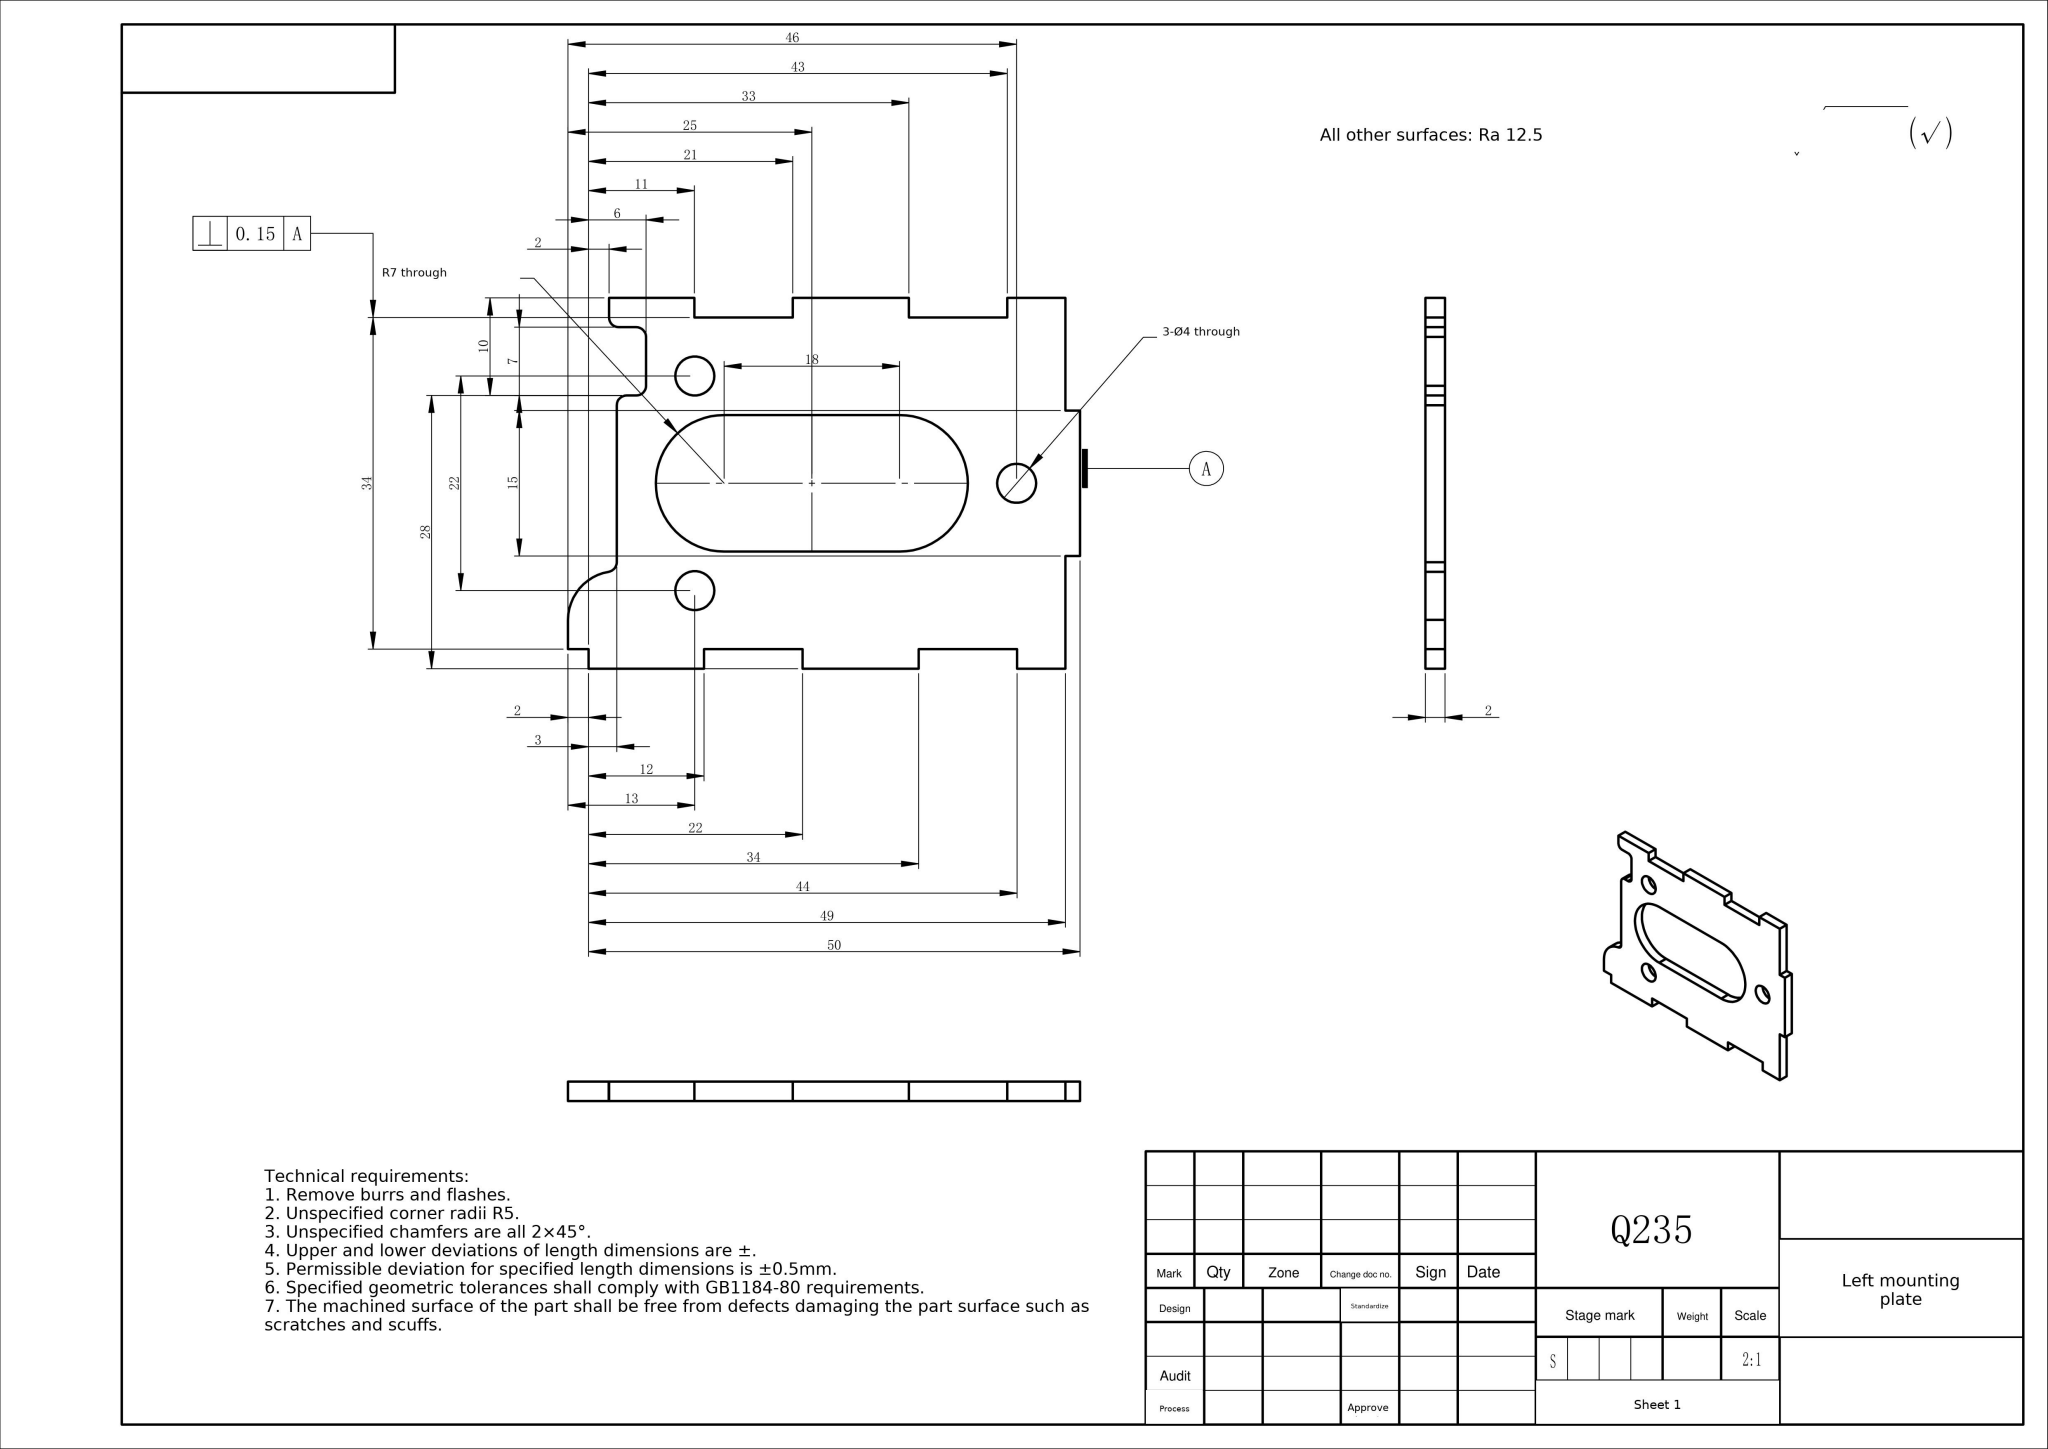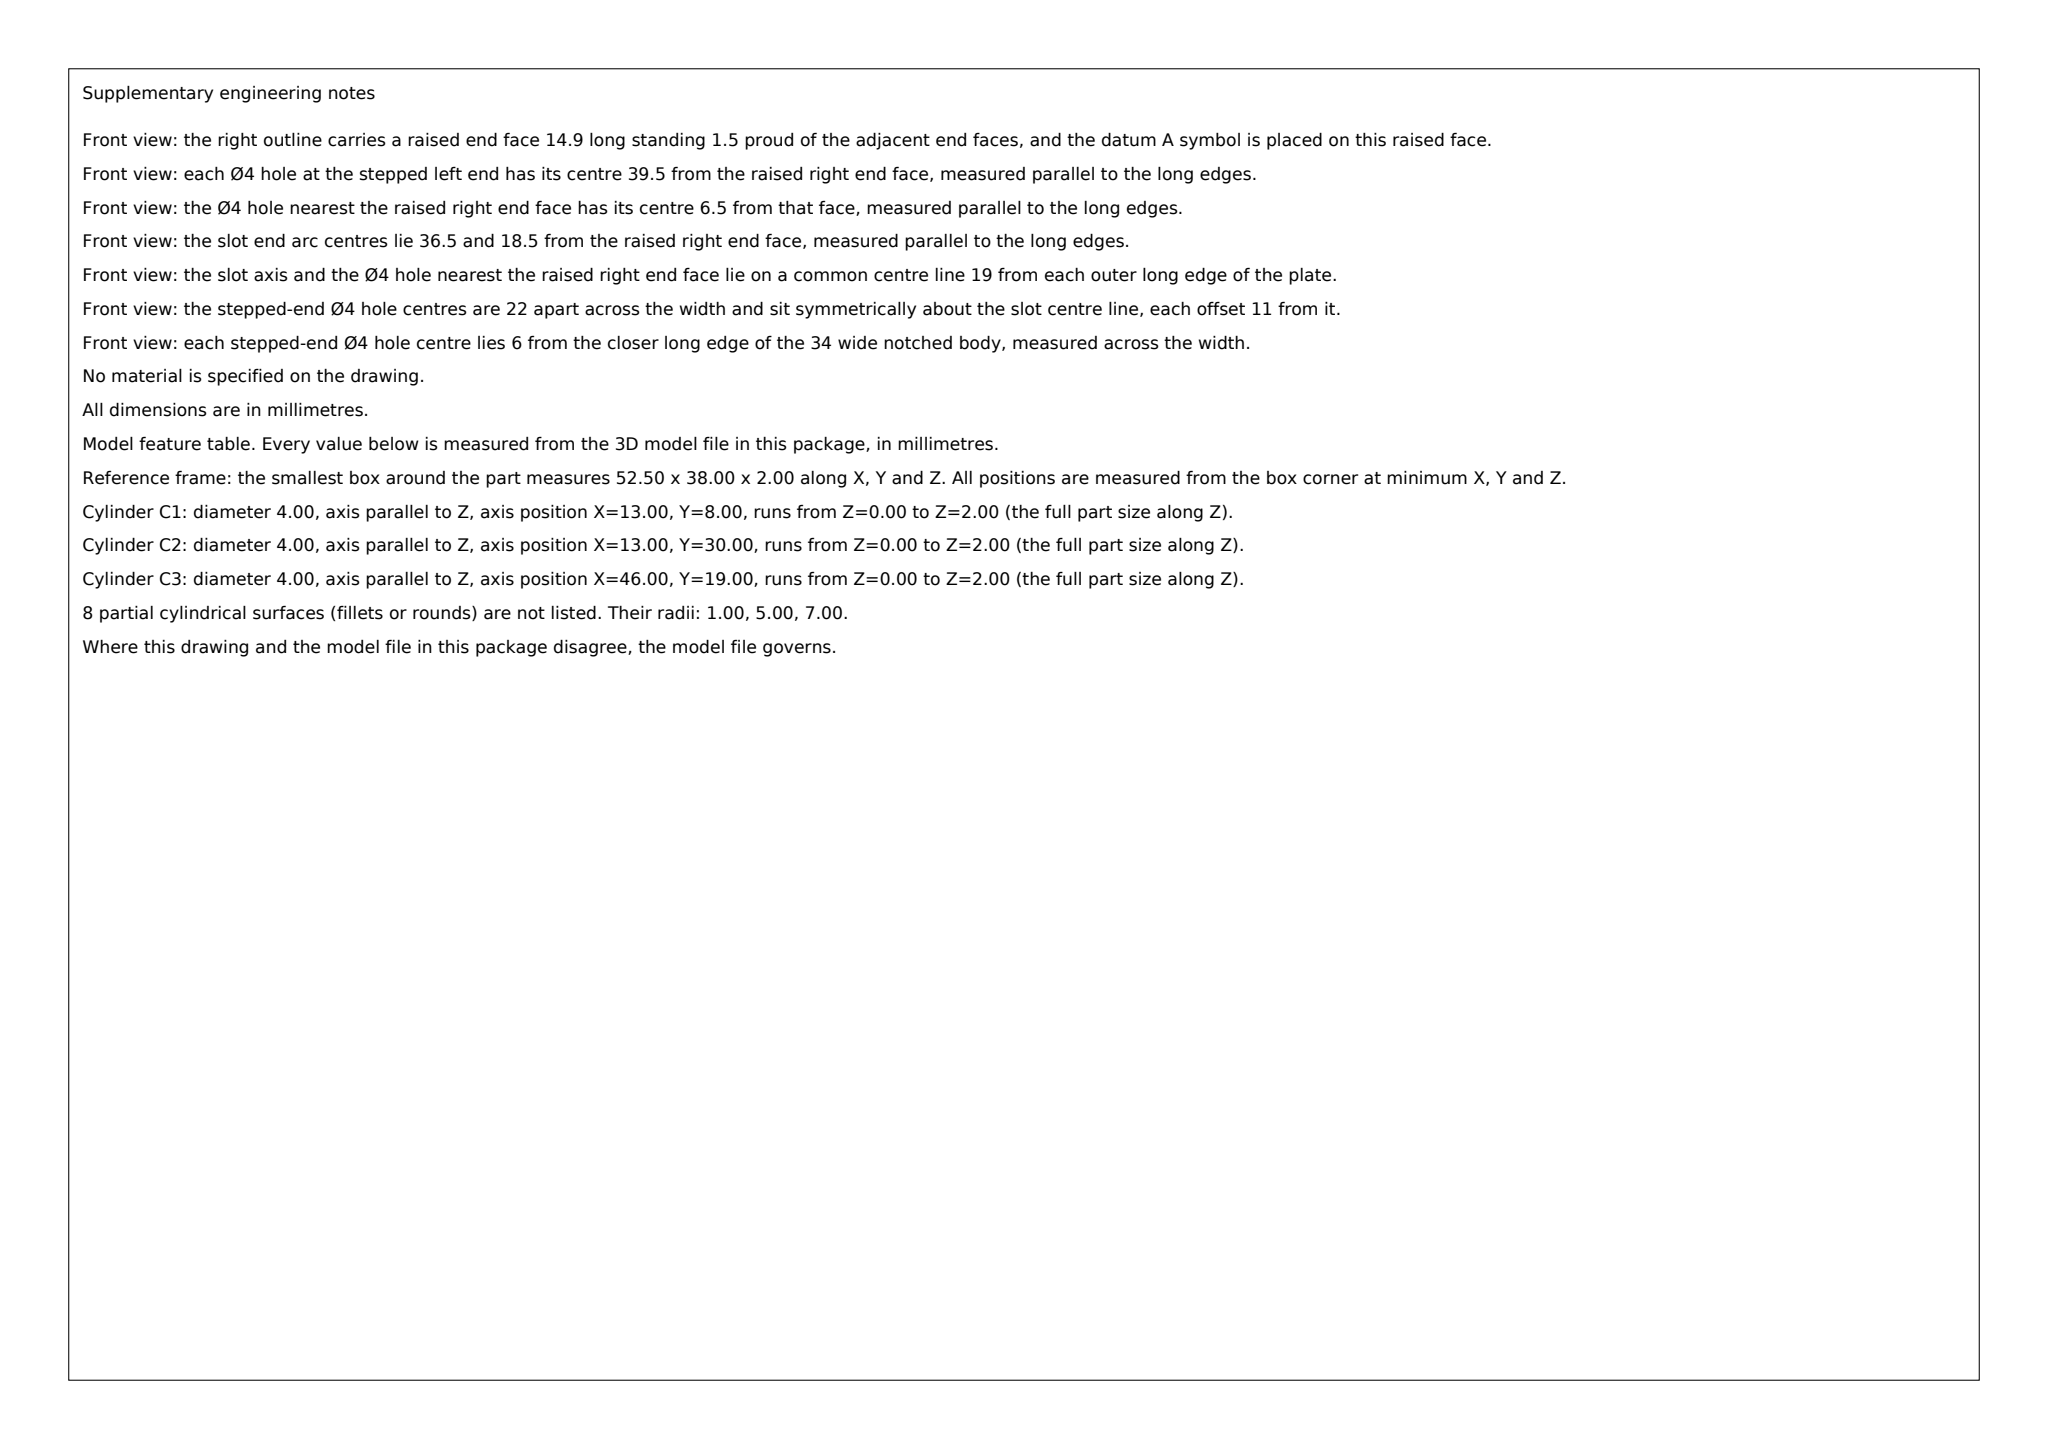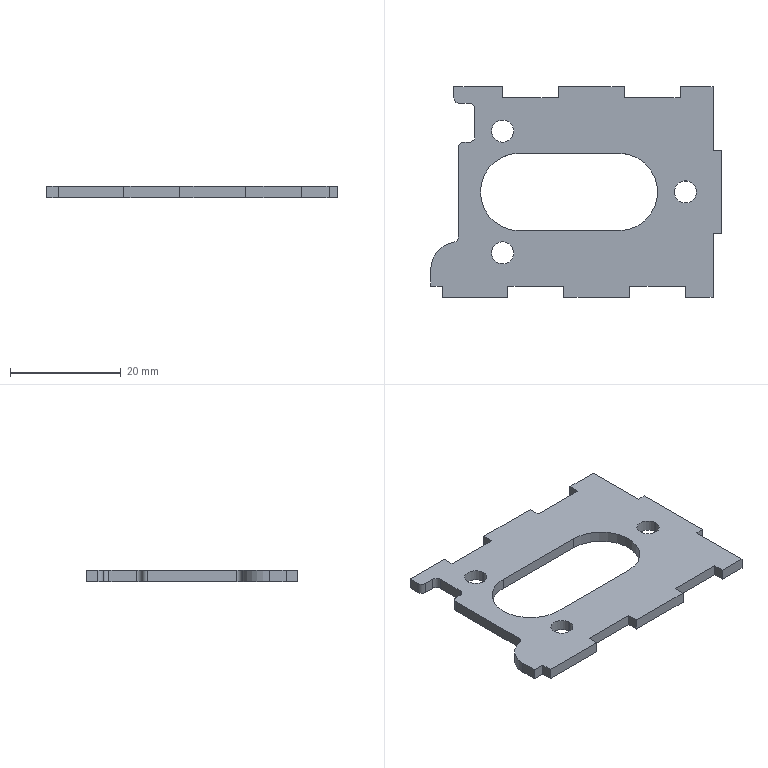Part | SolidWorks | mm | 1 solid | 50 faces | box 52.5 x 38 x 2 mm | volume 2536 mm3 | plane 35 | cylinder 15 | commonest cylinder face diameters 4 x6 2 x5 14 x3 10 x1
Drawing notes:
OVERALL LENGTH 52.5 INCL RH TAB (50 CHAIN + TAB PROJ) | from the solid: bbox_xyz x = 52.5; x-planes at 51 (body RH face) and 52.5 (tab end face)
OVERALL HEIGHT 38; TABS PROJ 2 BEYOND 34 TOP & BOT | from the solid: bbox_xyz y = 38; y-planes 0/2 and 36/38 bracket the 34 faces (y=2 to y=36)
RH TAB: 14.9 HIGH x 1.5 PROJ, FULL 2 THK, SYM ABT SLOT CL | from the solid: x-planes 51 to 52.5 = 1.5 proj; y-planes 11.55 & 26.45 = 14.9 high, sym abt y=19 (14 dia slot axes at y=19); z-planes 0 & 2